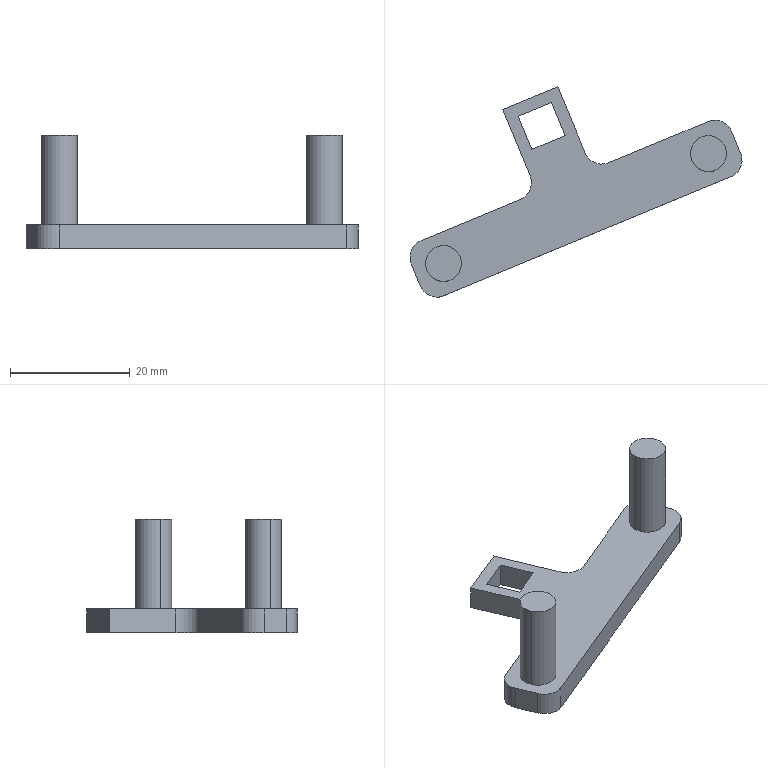Component | SolidWorks | Hanger-1 | 1 solid | 26 faces | box 55.57 x 35.2 x 19 mm | volume 3609 mm3 | plane 16 | cylinder 10 | commonest cylinder face diameters 6 x10
build123d program:
from build123d import *

# Parameters (mm, degrees)
SKETCH1_W           = 6
SKETCH1_H           = 6
BOSS_EXTRUDE1_DEPTH = 4
SKETCH2_R           = 3
BOSS_EXTRUDE2_DEPTH = 15


with BuildPart() as part:
    # Sketch1 → Boss-Extrude1 (new body)
    with BuildSketch(Plane.XY):
        with BuildLine():
            Line((-5.892, 5.811), (4.108, 5.811))
            Line((4.108, 5.811), (4.108, -4.189))
            Line((4.108, -4.189), (4.108, -6.189))
            ThreePointArc((4.108, -6.189), (4.987, -8.311), (7.108, -9.189))
            Line((7.108, -9.189), (25.108, -9.189))
            ThreePointArc((25.108, -9.189), (27.229, -10.068), (28.108, -12.189))
            Line((28.108, -12.189), (28.108, -16.189))
            ThreePointArc((28.108, -16.189), (27.229, -18.311), (25.108, -19.189))
            Line((25.108, -19.189), (-26.892, -19.189))
            ThreePointArc((-26.892, -19.189), (-29.013, -18.311), (-29.892, -16.189))
            Line((-29.892, -16.189), (-29.892, -12.189))
            ThreePointArc((-29.892, -12.189), (-29.013, -10.068), (-26.892, -9.189))
            Line((-26.892, -9.189), (-8.892, -9.189))
            ThreePointArc((-8.892, -9.189), (-6.771, -8.311), (-5.892, -6.189))
            Line((-5.892, -6.189), (-5.892, -4.189))
            Line((-5.892, -4.189), (-5.892, 5.811))
        make_face()
        with Locations((-0.8919, 0.8108)):
            Rectangle(SKETCH1_W, SKETCH1_H, mode=Mode.SUBTRACT)
    extrude(amount=BOSS_EXTRUDE1_DEPTH)

    # Sketch2 → Boss-Extrude2 (add)
    with BuildSketch(Plane(origin=(0, 0, 0), x_dir=(-1, 0, 0), z_dir=(0, 0, -1))):
        with Locations((-23.108, -14.189)):
            Circle(SKETCH2_R)
        with Locations(Location((24.892, -14.189, 0), (0, 0, 180))):
            Circle(SKETCH2_R)
    extrude(amount=BOSS_EXTRUDE2_DEPTH)


solid = part.part

# Placed as in the assembly
solid = solid.moved(Location((19.638, 31.834, 352.846), (180, 0, 157.477)))
STEP:
#1=COLOUR_RGB('',0.7922,0.8196,0.9333);
#2=FILL_AREA_STYLE_COLOUR('',#1);
#3=FILL_AREA_STYLE('',(#2));
#4=SURFACE_STYLE_FILL_AREA(#3);
#5=SURFACE_SIDE_STYLE('',(#4));
#6=SURFACE_STYLE_USAGE(.BOTH.,#5);
#7=PRESENTATION_STYLE_ASSIGNMENT((#6));
#8=CARTESIAN_POINT('',(2.001,1.158,14.482));
#9=VERTEX_POINT('',#8);
#10=CARTESIAN_POINT('',(1.783,1.067,14.482));
#11=VERTEX_POINT('',#10);
#12=CARTESIAN_POINT('',(1.892,1.113,14.482));
#13=DIRECTION('',(-0.,-0.,1.));
#14=DIRECTION('',(-0.9237,-0.383,0.));
#15=AXIS2_PLACEMENT_3D('',#12,#13,#14);
#16=CIRCLE('',#15,0.1181);
#17=EDGE_CURVE('',#9,#11,#16,.T.);
#18=ORIENTED_EDGE('',*,*,#17,.F.);
#19=CARTESIAN_POINT('',(2.001,1.158,13.892));
#20=VERTEX_POINT('',#19);
#21=CARTESIAN_POINT('',(2.001,1.158,14.482));
#22=DIRECTION('',(0.,0.,-1.));
#23=VECTOR('',#22,39.37);
#24=LINE('',#21,#23);
#25=EDGE_CURVE('',#9,#20,#24,.T.);
#26=ORIENTED_EDGE('',*,*,#25,.T.);
#27=CARTESIAN_POINT('',(1.783,1.067,13.892));
#28=VERTEX_POINT('',#27);
#29=CARTESIAN_POINT('',(1.892,1.113,13.892));
#30=DIRECTION('',(-0.,-0.,1.));
#31=DIRECTION('',(-0.9237,-0.383,0.));
#32=AXIS2_PLACEMENT_3D('',#29,#30,#31);
#33=CIRCLE('',#32,0.1181);
#34=EDGE_CURVE('',#20,#28,#33,.T.);
#35=ORIENTED_EDGE('',*,*,#34,.T.);
#36=CARTESIAN_POINT('',(1.783,1.067,14.482));
#37=DIRECTION('',(0.,0.,-1.));
#38=VECTOR('',#37,39.37);
#39=LINE('',#36,#38);
#40=EDGE_CURVE('',#11,#28,#39,.T.);
#41=ORIENTED_EDGE('',*,*,#40,.F.);
#42=EDGE_LOOP('',(#18,#26,#35,#41));
#43=FACE_OUTER_BOUND('',#42,.T.);
#44=CARTESIAN_POINT('',(1.892,1.113,14.482));
#45=DIRECTION('',(0.,0.,-1.));
#46=DIRECTION('',(-0.9237,-0.383,0.));
#47=AXIS2_PLACEMENT_3D('',#44,#45,#46);
#48=CYLINDRICAL_SURFACE('',#47,0.1181);
#49=ADVANCED_FACE('',(#43),#48,.T.);
#50=CARTESIAN_POINT('',(0.2558,0.4341,14.482));
#51=VERTEX_POINT('',#50);
#52=CARTESIAN_POINT('',(0.03764,0.3436,14.482));
#53=VERTEX_POINT('',#52);
#54=CARTESIAN_POINT('',(0.1467,0.3888,14.482));
#55=DIRECTION('',(-0.,-0.,1.));
#56=DIRECTION('',(0.9237,0.383,0.));
#57=AXIS2_PLACEMENT_3D('',#54,#55,#56);
#58=CIRCLE('',#57,0.1181);
#59=EDGE_CURVE('',#51,#53,#58,.T.);
#60=ORIENTED_EDGE('',*,*,#59,.F.);
#61=CARTESIAN_POINT('',(0.2558,0.4341,13.892));
#62=VERTEX_POINT('',#61);
#63=CARTESIAN_POINT('',(0.2558,0.4341,14.482));
#64=DIRECTION('',(0.,0.,-1.));
#65=VECTOR('',#64,39.37);
#66=LINE('',#63,#65);
#67=EDGE_CURVE('',#51,#62,#66,.T.);
#68=ORIENTED_EDGE('',*,*,#67,.T.);
#69=CARTESIAN_POINT('',(0.03764,0.3436,13.892));
#70=VERTEX_POINT('',#69);
#71=CARTESIAN_POINT('',(0.1467,0.3888,13.892));
#72=DIRECTION('',(-0.,-0.,1.));
#73=DIRECTION('',(0.9237,0.383,0.));
#74=AXIS2_PLACEMENT_3D('',#71,#72,#73);
#75=CIRCLE('',#74,0.1181);
#76=EDGE_CURVE('',#62,#70,#75,.T.);
#77=ORIENTED_EDGE('',*,*,#76,.T.);
#78=CARTESIAN_POINT('',(0.03764,0.3436,14.482));
#79=DIRECTION('',(0.,0.,-1.));
#80=VECTOR('',#79,39.37);
#81=LINE('',#78,#80);
#82=EDGE_CURVE('',#53,#70,#81,.T.);
#83=ORIENTED_EDGE('',*,*,#82,.F.);
#84=EDGE_LOOP('',(#60,#68,#77,#83));
#85=FACE_OUTER_BOUND('',#84,.T.);
#86=CARTESIAN_POINT('',(0.1467,0.3888,14.482));
#87=DIRECTION('',(0.,0.,-1.));
#88=DIRECTION('',(-0.9237,-0.383,0.));
#89=AXIS2_PLACEMENT_3D('',#86,#87,#88);
#90=CYLINDRICAL_SURFACE('',#89,0.1181);
#91=ADVANCED_FACE('',(#85),#90,.T.);
#92=CARTESIAN_POINT('',(0.8998,1.553,13.734));
#93=VERTEX_POINT('',#92);
#94=CARTESIAN_POINT('',(1.081,1.117,13.734));
#95=VERTEX_POINT('',#94);
#96=CARTESIAN_POINT('',(0.8998,1.553,13.734));
#97=DIRECTION('',(0.383,-0.9237,0.));
#98=VECTOR('',#97,39.37);
#99=LINE('',#96,#98);
#100=EDGE_CURVE('',#93,#95,#99,.T.);
#101=ORIENTED_EDGE('',*,*,#100,.T.);
#102=CARTESIAN_POINT('',(1.235,1.053,13.734));
#103=VERTEX_POINT('',#102);
#104=CARTESIAN_POINT('',(1.19,1.162,13.734));
#105=DIRECTION('',(-0.,-0.,1.));
#106=DIRECTION('',(0.9237,0.383,0.));
#107=AXIS2_PLACEMENT_3D('',#104,#105,#106);
#108=CIRCLE('',#107,0.1181);
#109=EDGE_CURVE('',#95,#103,#108,.T.);
#110=ORIENTED_EDGE('',*,*,#109,.T.);
#111=CARTESIAN_POINT('',(1.89,1.325,13.734));
#112=VERTEX_POINT('',#111);
#113=CARTESIAN_POINT('',(1.235,1.053,13.734));
#114=DIRECTION('',(0.9237,0.383,0.));
#115=VECTOR('',#114,39.37);
#116=LINE('',#113,#115);
#117=EDGE_CURVE('',#103,#112,#116,.T.);
#118=ORIENTED_EDGE('',*,*,#117,.T.);
#119=CARTESIAN_POINT('',(2.044,1.261,13.734));
#120=VERTEX_POINT('',#119);
#121=CARTESIAN_POINT('',(1.935,1.216,13.734));
#122=DIRECTION('',(0.,0.,-1.));
#123=DIRECTION('',(-0.9237,-0.383,0.));
#124=AXIS2_PLACEMENT_3D('',#121,#122,#123);
#125=CIRCLE('',#124,0.1181);
#126=EDGE_CURVE('',#112,#120,#125,.T.);
#127=ORIENTED_EDGE('',*,*,#126,.T.);
#128=CARTESIAN_POINT('',(2.104,1.115,13.734));
#129=VERTEX_POINT('',#128);
#130=CARTESIAN_POINT('',(2.044,1.261,13.734));
#131=DIRECTION('',(0.383,-0.9237,0.));
#132=VECTOR('',#131,39.37);
#133=LINE('',#130,#132);
#134=EDGE_CURVE('',#120,#129,#133,.T.);
#135=ORIENTED_EDGE('',*,*,#134,.T.);
#136=CARTESIAN_POINT('',(2.041,0.961,13.734));
#137=VERTEX_POINT('',#136);
#138=CARTESIAN_POINT('',(1.995,1.07,13.734));
#139=DIRECTION('',(0.,0.,-1.));
#140=DIRECTION('',(-0.9237,-0.383,0.));
#141=AXIS2_PLACEMENT_3D('',#138,#139,#140);
#142=CIRCLE('',#141,0.1181);
#143=EDGE_CURVE('',#129,#137,#142,.T.);
#144=ORIENTED_EDGE('',*,*,#143,.T.);
#145=CARTESIAN_POINT('',(0.1494,0.1768,13.734));
#146=VERTEX_POINT('',#145);
#147=CARTESIAN_POINT('',(2.041,0.961,13.734));
#148=DIRECTION('',(-0.9237,-0.383,-0.));
#149=VECTOR('',#148,39.37);
#150=LINE('',#147,#149);
#151=EDGE_CURVE('',#137,#146,#150,.T.);
#152=ORIENTED_EDGE('',*,*,#151,.T.);
#153=CARTESIAN_POINT('',(-0.004933,0.2407,13.734));
#154=VERTEX_POINT('',#153);
#155=CARTESIAN_POINT('',(0.1042,0.2859,13.734));
#156=DIRECTION('',(0.,0.,-1.));
#157=DIRECTION('',(0.9237,0.383,0.));
#158=AXIS2_PLACEMENT_3D('',#155,#156,#157);
#159=CIRCLE('',#158,0.1181);
#160=EDGE_CURVE('',#146,#154,#159,.T.);
#161=ORIENTED_EDGE('',*,*,#160,.T.);
#162=CARTESIAN_POINT('',(-0.06526,0.3861,13.734));
#163=VERTEX_POINT('',#162);
#164=CARTESIAN_POINT('',(-0.06526,0.3861,13.734));
#165=DIRECTION('',(-0.383,0.9237,0.));
#166=VECTOR('',#165,39.37);
#167=LINE('',#164,#166);
#168=EDGE_CURVE('',#154,#163,#167,.T.);
#169=ORIENTED_EDGE('',*,*,#168,.T.);
#170=CARTESIAN_POINT('',(-0.001396,0.5405,13.734));
#171=VERTEX_POINT('',#170);
#172=CARTESIAN_POINT('',(0.04385,0.4314,13.734));
#173=DIRECTION('',(0.,0.,-1.));
#174=DIRECTION('',(-0.9237,-0.383,0.));
#175=AXIS2_PLACEMENT_3D('',#172,#173,#174);
#176=CIRCLE('',#175,0.1181);
#177=EDGE_CURVE('',#163,#171,#176,.T.);
#178=ORIENTED_EDGE('',*,*,#177,.T.);
#179=CARTESIAN_POINT('',(0.6532,0.8119,13.734));
#180=VERTEX_POINT('',#179);
#181=CARTESIAN_POINT('',(0.6532,0.8119,13.734));
#182=DIRECTION('',(0.9237,0.383,0.));
#183=VECTOR('',#182,39.37);
#184=LINE('',#181,#183);
#185=EDGE_CURVE('',#171,#180,#184,.T.);
#186=ORIENTED_EDGE('',*,*,#185,.T.);
#187=CARTESIAN_POINT('',(0.7171,0.9663,13.734));
#188=VERTEX_POINT('',#187);
#189=CARTESIAN_POINT('',(0.608,0.921,13.734));
#190=DIRECTION('',(-0.,-0.,1.));
#191=DIRECTION('',(-0.9237,-0.383,0.));
#192=AXIS2_PLACEMENT_3D('',#189,#190,#191);
#193=CIRCLE('',#192,0.1181);
#194=EDGE_CURVE('',#180,#188,#193,.T.);
#195=ORIENTED_EDGE('',*,*,#194,.T.);
#196=CARTESIAN_POINT('',(0.5361,1.403,13.734));
#197=VERTEX_POINT('',#196);
#198=CARTESIAN_POINT('',(0.6869,1.039,13.734));
#199=DIRECTION('',(-0.383,0.9237,-0.));
#200=VECTOR('',#199,39.37);
#201=LINE('',#198,#200);
#202=EDGE_CURVE('',#188,#197,#201,.T.);
#203=ORIENTED_EDGE('',*,*,#202,.T.);
#204=CARTESIAN_POINT('',(0.8998,1.553,13.734));
#205=DIRECTION('',(0.9237,0.383,0.));
#206=VECTOR('',#205,39.37);
#207=LINE('',#204,#206);
#208=EDGE_CURVE('',#197,#93,#207,.T.);
#209=ORIENTED_EDGE('',*,*,#208,.T.);
#210=EDGE_LOOP('',(#101,#110,#118,#127,#135,#144,#152,#161,#169,#178,#186,#195,#203,#209));
#211=FACE_OUTER_BOUND('',#210,.T.);
#212=CARTESIAN_POINT('',(0.8572,1.451,13.734));
#213=VERTEX_POINT('',#212);
#214=CARTESIAN_POINT('',(0.9477,1.232,13.734));
#215=VERTEX_POINT('',#214);
#216=CARTESIAN_POINT('',(0.8572,1.451,13.734));
#217=DIRECTION('',(0.383,-0.9237,-0.));
#218=VECTOR('',#217,39.37);
#219=LINE('',#216,#218);
#220=EDGE_CURVE('',#213,#215,#219,.T.);
#221=ORIENTED_EDGE('',*,*,#220,.F.);
#222=CARTESIAN_POINT('',(0.639,1.36,13.734));
#223=VERTEX_POINT('',#222);
#224=CARTESIAN_POINT('',(0.8572,1.451,13.734));
#225=DIRECTION('',(0.9237,0.383,0.));
#226=VECTOR('',#225,39.37);
#227=LINE('',#224,#226);
#228=EDGE_CURVE('',#223,#213,#227,.T.);
#229=ORIENTED_EDGE('',*,*,#228,.F.);
#230=CARTESIAN_POINT('',(0.7295,1.142,13.734));
#231=VERTEX_POINT('',#230);
#232=CARTESIAN_POINT('',(0.639,1.36,13.734));
#233=DIRECTION('',(-0.383,0.9237,0.));
#234=VECTOR('',#233,39.37);
#235=LINE('',#232,#234);
#236=EDGE_CURVE('',#231,#223,#235,.T.);
#237=ORIENTED_EDGE('',*,*,#236,.F.);
#238=CARTESIAN_POINT('',(0.9477,1.232,13.734));
#239=DIRECTION('',(-0.9237,-0.383,-0.));
#240=VECTOR('',#239,39.37);
#241=LINE('',#238,#240);
#242=EDGE_CURVE('',#215,#231,#241,.T.);
#243=ORIENTED_EDGE('',*,*,#242,.F.);
#244=EDGE_LOOP('',(#221,#229,#237,#243));
#245=FACE_BOUND('',#244,.T.);
#246=CARTESIAN_POINT('',(1.19,1.162,13.734));
#247=DIRECTION('',(-0.,-0.,1.));
#248=DIRECTION('',(0.9237,0.383,0.));
#249=AXIS2_PLACEMENT_3D('',#246,#247,#248);
#250=PLANE('',#249);
#251=ADVANCED_FACE('',(#211,#245),#250,.F.);
#252=CARTESIAN_POINT('',(1.892,1.113,13.892));
#253=DIRECTION('',(-0.,-0.,1.));
#254=DIRECTION('',(-0.9237,-0.383,0.));
#255=AXIS2_PLACEMENT_3D('',#252,#253,#254);
#256=CIRCLE('',#255,0.1181);
#257=EDGE_CURVE('',#28,#20,#256,.T.);
#258=ORIENTED_EDGE('',*,*,#257,.F.);
#259=ORIENTED_EDGE('',*,*,#34,.F.);
#260=EDGE_LOOP('',(#258,#259));
#261=FACE_BOUND('',#260,.T.);
#262=CARTESIAN_POINT('',(0.1467,0.3888,13.892));
#263=DIRECTION('',(-0.,-0.,1.));
#264=DIRECTION('',(0.9237,0.383,0.));
#265=AXIS2_PLACEMENT_3D('',#262,#263,#264);
#266=CIRCLE('',#265,0.1181);
#267=EDGE_CURVE('',#70,#62,#266,.T.);
#268=ORIENTED_EDGE('',*,*,#267,.F.);
#269=ORIENTED_EDGE('',*,*,#76,.F.);
#270=EDGE_LOOP('',(#268,#269));
#271=FACE_BOUND('',#270,.T.);
#272=CARTESIAN_POINT('',(0.8998,1.553,13.892));
#273=VERTEX_POINT('',#272);
#274=CARTESIAN_POINT('',(1.081,1.117,13.892));
#275=VERTEX_POINT('',#274);
#276=CARTESIAN_POINT('',(1.051,1.19,13.892));
#277=DIRECTION('',(0.383,-0.9237,-0.));
#278=VECTOR('',#277,39.37);
#279=LINE('',#276,#278);
#280=EDGE_CURVE('',#273,#275,#279,.T.);
#281=ORIENTED_EDGE('',*,*,#280,.F.);
#282=CARTESIAN_POINT('',(0.5361,1.403,13.892));
#283=VERTEX_POINT('',#282);
#284=CARTESIAN_POINT('',(0.8998,1.553,13.892));
#285=DIRECTION('',(0.9237,0.383,0.));
#286=VECTOR('',#285,39.37);
#287=LINE('',#284,#286);
#288=EDGE_CURVE('',#283,#273,#287,.T.);
#289=ORIENTED_EDGE('',*,*,#288,.F.);
#290=CARTESIAN_POINT('',(0.7171,0.9663,13.892));
#291=VERTEX_POINT('',#290);
#292=CARTESIAN_POINT('',(0.5361,1.403,13.892));
#293=DIRECTION('',(-0.383,0.9237,0.));
#294=VECTOR('',#293,39.37);
#295=LINE('',#292,#294);
#296=EDGE_CURVE('',#291,#283,#295,.T.);
#297=ORIENTED_EDGE('',*,*,#296,.F.);
#298=CARTESIAN_POINT('',(0.6532,0.8119,13.892));
#299=VERTEX_POINT('',#298);
#300=CARTESIAN_POINT('',(0.608,0.921,13.892));
#301=DIRECTION('',(-0.,-0.,1.));
#302=DIRECTION('',(-0.9237,-0.383,0.));
#303=AXIS2_PLACEMENT_3D('',#300,#301,#302);
#304=CIRCLE('',#303,0.1181);
#305=EDGE_CURVE('',#299,#291,#304,.T.);
#306=ORIENTED_EDGE('',*,*,#305,.F.);
#307=CARTESIAN_POINT('',(-0.001396,0.5405,13.892));
#308=VERTEX_POINT('',#307);
#309=CARTESIAN_POINT('',(0.6532,0.8119,13.892));
#310=DIRECTION('',(0.9237,0.383,0.));
#311=VECTOR('',#310,39.37);
#312=LINE('',#309,#311);
#313=EDGE_CURVE('',#308,#299,#312,.T.);
#314=ORIENTED_EDGE('',*,*,#313,.F.);
#315=CARTESIAN_POINT('',(-0.06526,0.3861,13.892));
#316=VERTEX_POINT('',#315);
#317=CARTESIAN_POINT('',(0.04385,0.4314,13.892));
#318=DIRECTION('',(0.,0.,-1.));
#319=DIRECTION('',(-0.9237,-0.383,0.));
#320=AXIS2_PLACEMENT_3D('',#317,#318,#319);
#321=CIRCLE('',#320,0.1181);
#322=EDGE_CURVE('',#316,#308,#321,.T.);
#323=ORIENTED_EDGE('',*,*,#322,.F.);
#324=CARTESIAN_POINT('',(-0.004933,0.2407,13.892));
#325=VERTEX_POINT('',#324);
#326=CARTESIAN_POINT('',(-0.06526,0.3861,13.892));
#327=DIRECTION('',(-0.383,0.9237,0.));
#328=VECTOR('',#327,39.37);
#329=LINE('',#326,#328);
#330=EDGE_CURVE('',#325,#316,#329,.T.);
#331=ORIENTED_EDGE('',*,*,#330,.F.);
#332=CARTESIAN_POINT('',(0.1494,0.1768,13.892));
#333=VERTEX_POINT('',#332);
#334=CARTESIAN_POINT('',(0.1042,0.2859,13.892));
#335=DIRECTION('',(0.,0.,-1.));
#336=DIRECTION('',(0.9237,0.383,0.));
#337=AXIS2_PLACEMENT_3D('',#334,#335,#336);
#338=CIRCLE('',#337,0.1181);
#339=EDGE_CURVE('',#333,#325,#338,.T.);
#340=ORIENTED_EDGE('',*,*,#339,.F.);
#341=CARTESIAN_POINT('',(2.041,0.961,13.892));
#342=VERTEX_POINT('',#341);
#343=CARTESIAN_POINT('',(2.041,0.961,13.892));
#344=DIRECTION('',(-0.9237,-0.383,-0.));
#345=VECTOR('',#344,39.37);
#346=LINE('',#343,#345);
#347=EDGE_CURVE('',#342,#333,#346,.T.);
#348=ORIENTED_EDGE('',*,*,#347,.F.);
#349=CARTESIAN_POINT('',(2.104,1.115,13.892));
#350=VERTEX_POINT('',#349);
#351=CARTESIAN_POINT('',(1.995,1.07,13.892));
#352=DIRECTION('',(0.,0.,-1.));
#353=DIRECTION('',(-0.9237,-0.383,0.));
#354=AXIS2_PLACEMENT_3D('',#351,#352,#353);
#355=CIRCLE('',#354,0.1181);
#356=EDGE_CURVE('',#350,#342,#355,.T.);
#357=ORIENTED_EDGE('',*,*,#356,.F.);
#358=CARTESIAN_POINT('',(2.044,1.261,13.892));
#359=VERTEX_POINT('',#358);
#360=CARTESIAN_POINT('',(2.044,1.261,13.892));
#361=DIRECTION('',(0.383,-0.9237,0.));
#362=VECTOR('',#361,39.37);
#363=LINE('',#360,#362);
#364=EDGE_CURVE('',#359,#350,#363,.T.);
#365=ORIENTED_EDGE('',*,*,#364,.F.);
#366=CARTESIAN_POINT('',(1.89,1.325,13.892));
#367=VERTEX_POINT('',#366);
#368=CARTESIAN_POINT('',(1.935,1.216,13.892));
#369=DIRECTION('',(0.,0.,-1.));
#370=DIRECTION('',(-0.9237,-0.383,0.));
#371=AXIS2_PLACEMENT_3D('',#368,#369,#370);
#372=CIRCLE('',#371,0.1181);
#373=EDGE_CURVE('',#367,#359,#372,.T.);
#374=ORIENTED_EDGE('',*,*,#373,.F.);
#375=CARTESIAN_POINT('',(1.235,1.053,13.892));
#376=VERTEX_POINT('',#375);
#377=CARTESIAN_POINT('',(1.235,1.053,13.892));
#378=DIRECTION('',(0.9237,0.383,0.));
#379=VECTOR('',#378,39.37);
#380=LINE('',#377,#379);
#381=EDGE_CURVE('',#376,#367,#380,.T.);
#382=ORIENTED_EDGE('',*,*,#381,.F.);
#383=CARTESIAN_POINT('',(1.19,1.162,13.892));
#384=DIRECTION('',(-0.,-0.,1.));
#385=DIRECTION('',(0.9237,0.383,0.));
#386=AXIS2_PLACEMENT_3D('',#383,#384,#385);
#387=CIRCLE('',#386,0.1181);
#388=EDGE_CURVE('',#275,#376,#387,.T.);
#389=ORIENTED_EDGE('',*,*,#388,.F.);
#390=EDGE_LOOP('',(#281,#289,#297,#306,#314,#323,#331,#340,#348,#357,#365,#374,#382,#389));
#391=FACE_OUTER_BOUND('',#390,.T.);
#392=CARTESIAN_POINT('',(0.639,1.36,13.892));
#393=VERTEX_POINT('',#392);
#394=CARTESIAN_POINT('',(0.8572,1.451,13.892));
#395=VERTEX_POINT('',#394);
#396=CARTESIAN_POINT('',(0.8572,1.451,13.892));
#397=DIRECTION('',(0.9237,0.383,0.));
#398=VECTOR('',#397,39.37);
#399=LINE('',#396,#398);
#400=EDGE_CURVE('',#393,#395,#399,.T.);
#401=ORIENTED_EDGE('',*,*,#400,.T.);
#402=CARTESIAN_POINT('',(0.9477,1.232,13.892));
#403=VERTEX_POINT('',#402);
#404=CARTESIAN_POINT('',(0.8572,1.451,13.892));
#405=DIRECTION('',(0.383,-0.9237,-0.));
#406=VECTOR('',#405,39.37);
#407=LINE('',#404,#406);
#408=EDGE_CURVE('',#395,#403,#407,.T.);
#409=ORIENTED_EDGE('',*,*,#408,.T.);
#410=CARTESIAN_POINT('',(0.7295,1.142,13.892));
#411=VERTEX_POINT('',#410);
#412=CARTESIAN_POINT('',(0.9477,1.232,13.892));
#413=DIRECTION('',(-0.9237,-0.383,-0.));
#414=VECTOR('',#413,39.37);
#415=LINE('',#412,#414);
#416=EDGE_CURVE('',#403,#411,#415,.T.);
#417=ORIENTED_EDGE('',*,*,#416,.T.);
#418=CARTESIAN_POINT('',(0.639,1.36,13.892));
#419=DIRECTION('',(-0.383,0.9237,0.));
#420=VECTOR('',#419,39.37);
#421=LINE('',#418,#420);
#422=EDGE_CURVE('',#411,#393,#421,.T.);
#423=ORIENTED_EDGE('',*,*,#422,.T.);
#424=EDGE_LOOP('',(#401,#409,#417,#423));
#425=FACE_BOUND('',#424,.T.);
#426=CARTESIAN_POINT('',(1.19,1.162,13.892));
#427=DIRECTION('',(-0.,-0.,1.));
#428=DIRECTION('',(0.9237,0.383,0.));
#429=AXIS2_PLACEMENT_3D('',#426,#427,#428);
#430=PLANE('',#429);
#431=ADVANCED_FACE('',(#261,#271,#391,#425),#430,.T.);
#432=ORIENTED_EDGE('',*,*,#280,.T.);
#433=CARTESIAN_POINT('',(1.081,1.117,13.734));
#434=DIRECTION('',(-0.,-0.,1.));
#435=VECTOR('',#434,39.37);
#436=LINE('',#433,#435);
#437=EDGE_CURVE('',#95,#275,#436,.T.);
#438=ORIENTED_EDGE('',*,*,#437,.F.);
#439=ORIENTED_EDGE('',*,*,#100,.F.);
#440=CARTESIAN_POINT('',(0.8998,1.553,13.734));
#441=DIRECTION('',(-0.,-0.,1.));
#442=VECTOR('',#441,39.37);
#443=LINE('',#440,#442);
#444=EDGE_CURVE('',#93,#273,#443,.T.);
#445=ORIENTED_EDGE('',*,*,#444,.T.);
#446=EDGE_LOOP('',(#432,#438,#439,#445));
#447=FACE_OUTER_BOUND('',#446,.T.);
#448=CARTESIAN_POINT('',(1.051,1.19,13.734));
#449=DIRECTION('',(-0.9237,-0.383,-0.));
#450=DIRECTION('',(-0.383,0.9237,0.));
#451=AXIS2_PLACEMENT_3D('',#448,#449,#450);
#452=PLANE('',#451);
#453=ADVANCED_FACE('',(#447),#452,.F.);
#454=ORIENTED_EDGE('',*,*,#388,.T.);
#455=CARTESIAN_POINT('',(1.235,1.053,13.734));
#456=DIRECTION('',(-0.,-0.,1.));
#457=VECTOR('',#456,39.37);
#458=LINE('',#455,#457);
#459=EDGE_CURVE('',#103,#376,#458,.T.);
#460=ORIENTED_EDGE('',*,*,#459,.F.);
#461=ORIENTED_EDGE('',*,*,#109,.F.);
#462=ORIENTED_EDGE('',*,*,#437,.T.);
#463=EDGE_LOOP('',(#454,#460,#461,#462));
#464=FACE_OUTER_BOUND('',#463,.T.);
#465=CARTESIAN_POINT('',(1.19,1.162,13.734));
#466=DIRECTION('',(-0.,-0.,1.));
#467=DIRECTION('',(0.9237,0.383,0.));
#468=AXIS2_PLACEMENT_3D('',#465,#466,#467);
#469=CYLINDRICAL_SURFACE('',#468,0.1181);
#470=ADVANCED_FACE('',(#464),#469,.F.);
#471=ORIENTED_EDGE('',*,*,#381,.T.);
#472=CARTESIAN_POINT('',(1.89,1.325,13.734));
#473=DIRECTION('',(-0.,-0.,1.));
#474=VECTOR('',#473,39.37);
#475=LINE('',#472,#474);
#476=EDGE_CURVE('',#112,#367,#475,.T.);
#477=ORIENTED_EDGE('',*,*,#476,.F.);
#478=ORIENTED_EDGE('',*,*,#117,.F.);
#479=ORIENTED_EDGE('',*,*,#459,.T.);
#480=EDGE_LOOP('',(#471,#477,#478,#479));
#481=FACE_OUTER_BOUND('',#480,.T.);
#482=CARTESIAN_POINT('',(1.235,1.053,13.734));
#483=DIRECTION('',(0.383,-0.9237,-0.));
#484=DIRECTION('',(-0.9237,-0.383,-0.));
#485=AXIS2_PLACEMENT_3D('',#482,#483,#484);
#486=PLANE('',#485);
#487=ADVANCED_FACE('',(#481),#486,.F.);
#488=ORIENTED_EDGE('',*,*,#373,.T.);
#489=CARTESIAN_POINT('',(2.044,1.261,13.734));
#490=DIRECTION('',(-0.,-0.,1.));
#491=VECTOR('',#490,39.37);
#492=LINE('',#489,#491);
#493=EDGE_CURVE('',#120,#359,#492,.T.);
#494=ORIENTED_EDGE('',*,*,#493,.F.);
#495=ORIENTED_EDGE('',*,*,#126,.F.);
#496=ORIENTED_EDGE('',*,*,#476,.T.);
#497=EDGE_LOOP('',(#488,#494,#495,#496));
#498=FACE_OUTER_BOUND('',#497,.T.);
#499=CARTESIAN_POINT('',(1.935,1.216,13.734));
#500=DIRECTION('',(-0.,-0.,1.));
#501=DIRECTION('',(0.9237,0.383,0.));
#502=AXIS2_PLACEMENT_3D('',#499,#500,#501);
#503=CYLINDRICAL_SURFACE('',#502,0.1181);
#504=ADVANCED_FACE('',(#498),#503,.T.);
#505=ORIENTED_EDGE('',*,*,#364,.T.);
#506=CARTESIAN_POINT('',(2.104,1.115,13.734));
#507=DIRECTION('',(-0.,-0.,1.));
#508=VECTOR('',#507,39.37);
#509=LINE('',#506,#508);
#510=EDGE_CURVE('',#129,#350,#509,.T.);
#511=ORIENTED_EDGE('',*,*,#510,.F.);
#512=ORIENTED_EDGE('',*,*,#134,.F.);
#513=ORIENTED_EDGE('',*,*,#493,.T.);
#514=EDGE_LOOP('',(#505,#511,#512,#513));
#515=FACE_OUTER_BOUND('',#514,.T.);
#516=CARTESIAN_POINT('',(2.044,1.261,13.734));
#517=DIRECTION('',(-0.9237,-0.383,-0.));
#518=DIRECTION('',(-0.,-0.,1.));
#519=AXIS2_PLACEMENT_3D('',#516,#517,#518);
#520=PLANE('',#519);
#521=ADVANCED_FACE('',(#515),#520,.F.);
#522=ORIENTED_EDGE('',*,*,#356,.T.);
#523=CARTESIAN_POINT('',(2.041,0.961,13.734));
#524=DIRECTION('',(-0.,-0.,1.));
#525=VECTOR('',#524,39.37);
#526=LINE('',#523,#525);
#527=EDGE_CURVE('',#137,#342,#526,.T.);
#528=ORIENTED_EDGE('',*,*,#527,.F.);
#529=ORIENTED_EDGE('',*,*,#143,.F.);
#530=ORIENTED_EDGE('',*,*,#510,.T.);
#531=EDGE_LOOP('',(#522,#528,#529,#530));
#532=FACE_OUTER_BOUND('',#531,.T.);
#533=CARTESIAN_POINT('',(1.995,1.07,13.734));
#534=DIRECTION('',(-0.,-0.,1.));
#535=DIRECTION('',(0.9237,0.383,0.));
#536=AXIS2_PLACEMENT_3D('',#533,#534,#535);
#537=CYLINDRICAL_SURFACE('',#536,0.1181);
#538=ADVANCED_FACE('',(#532),#537,.T.);
#539=ORIENTED_EDGE('',*,*,#347,.T.);
#540=CARTESIAN_POINT('',(0.1494,0.1768,13.734));
#541=DIRECTION('',(-0.,-0.,1.));
#542=VECTOR('',#541,39.37);
#543=LINE('',#540,#542);
#544=EDGE_CURVE('',#146,#333,#543,.T.);
#545=ORIENTED_EDGE('',*,*,#544,.F.);
#546=ORIENTED_EDGE('',*,*,#151,.F.);
#547=ORIENTED_EDGE('',*,*,#527,.T.);
#548=EDGE_LOOP('',(#539,#545,#546,#547));
#549=FACE_OUTER_BOUND('',#548,.T.);
#550=CARTESIAN_POINT('',(2.041,0.961,13.734));
#551=DIRECTION('',(-0.383,0.9237,0.));
#552=DIRECTION('',(0.,0.,-1.));
#553=AXIS2_PLACEMENT_3D('',#550,#551,#552);
#554=PLANE('',#553);
#555=ADVANCED_FACE('',(#549),#554,.F.);
#556=ORIENTED_EDGE('',*,*,#339,.T.);
#557=CARTESIAN_POINT('',(-0.004933,0.2407,13.734));
#558=DIRECTION('',(-0.,-0.,1.));
#559=VECTOR('',#558,39.37);
#560=LINE('',#557,#559);
#561=EDGE_CURVE('',#154,#325,#560,.T.);
#562=ORIENTED_EDGE('',*,*,#561,.F.);
#563=ORIENTED_EDGE('',*,*,#160,.F.);
#564=ORIENTED_EDGE('',*,*,#544,.T.);
#565=EDGE_LOOP('',(#556,#562,#563,#564));
#566=FACE_OUTER_BOUND('',#565,.T.);
#567=CARTESIAN_POINT('',(0.1042,0.2859,13.734));
#568=DIRECTION('',(-0.,-0.,1.));
#569=DIRECTION('',(0.9237,0.383,0.));
#570=AXIS2_PLACEMENT_3D('',#567,#568,#569);
#571=CYLINDRICAL_SURFACE('',#570,0.1181);
#572=ADVANCED_FACE('',(#566),#571,.T.);
#573=ORIENTED_EDGE('',*,*,#330,.T.);
#574=CARTESIAN_POINT('',(-0.06526,0.3861,13.734));
#575=DIRECTION('',(-0.,-0.,1.));
#576=VECTOR('',#575,39.37);
#577=LINE('',#574,#576);
#578=EDGE_CURVE('',#163,#316,#577,.T.);
#579=ORIENTED_EDGE('',*,*,#578,.F.);
#580=ORIENTED_EDGE('',*,*,#168,.F.);
#581=ORIENTED_EDGE('',*,*,#561,.T.);
#582=EDGE_LOOP('',(#573,#579,#580,#581));
#583=FACE_OUTER_BOUND('',#582,.T.);
#584=CARTESIAN_POINT('',(-0.06526,0.3861,13.734));
#585=DIRECTION('',(0.9237,0.383,0.));
#586=DIRECTION('',(0.,0.,-1.));
#587=AXIS2_PLACEMENT_3D('',#584,#585,#586);
#588=PLANE('',#587);
#589=ADVANCED_FACE('',(#583),#588,.F.);
#590=ORIENTED_EDGE('',*,*,#322,.T.);
#591=CARTESIAN_POINT('',(-0.001396,0.5405,13.734));
#592=DIRECTION('',(-0.,-0.,1.));
#593=VECTOR('',#592,39.37);
#594=LINE('',#591,#593);
#595=EDGE_CURVE('',#171,#308,#594,.T.);
#596=ORIENTED_EDGE('',*,*,#595,.F.);
#597=ORIENTED_EDGE('',*,*,#177,.F.);
#598=ORIENTED_EDGE('',*,*,#578,.T.);
#599=EDGE_LOOP('',(#590,#596,#597,#598));
#600=FACE_OUTER_BOUND('',#599,.T.);
#601=CARTESIAN_POINT('',(0.04385,0.4314,13.734));
#602=DIRECTION('',(-0.,-0.,1.));
#603=DIRECTION('',(0.9237,0.383,0.));
#604=AXIS2_PLACEMENT_3D('',#601,#602,#603);
#605=CYLINDRICAL_SURFACE('',#604,0.1181);
#606=ADVANCED_FACE('',(#600),#605,.T.);
#607=ORIENTED_EDGE('',*,*,#313,.T.);
#608=CARTESIAN_POINT('',(0.6532,0.8119,13.734));
#609=DIRECTION('',(-0.,-0.,1.));
#610=VECTOR('',#609,39.37);
#611=LINE('',#608,#610);
#612=EDGE_CURVE('',#180,#299,#611,.T.);
#613=ORIENTED_EDGE('',*,*,#612,.F.);
#614=ORIENTED_EDGE('',*,*,#185,.F.);
#615=ORIENTED_EDGE('',*,*,#595,.T.);
#616=EDGE_LOOP('',(#607,#613,#614,#615));
#617=FACE_OUTER_BOUND('',#616,.T.);
#618=CARTESIAN_POINT('',(0.6532,0.8119,13.734));
#619=DIRECTION('',(0.383,-0.9237,0.));
#620=DIRECTION('',(-0.9237,-0.383,-0.));
#621=AXIS2_PLACEMENT_3D('',#618,#619,#620);
#622=PLANE('',#621);
#623=ADVANCED_FACE('',(#617),#622,.F.);
#624=ORIENTED_EDGE('',*,*,#305,.T.);
#625=CARTESIAN_POINT('',(0.7171,0.9663,13.734));
#626=DIRECTION('',(-0.,-0.,1.));
#627=VECTOR('',#626,39.37);
#628=LINE('',#625,#627);
#629=EDGE_CURVE('',#188,#291,#628,.T.);
#630=ORIENTED_EDGE('',*,*,#629,.F.);
#631=ORIENTED_EDGE('',*,*,#194,.F.);
#632=ORIENTED_EDGE('',*,*,#612,.T.);
#633=EDGE_LOOP('',(#624,#630,#631,#632));
#634=FACE_OUTER_BOUND('',#633,.T.);
#635=CARTESIAN_POINT('',(0.608,0.921,13.734));
#636=DIRECTION('',(-0.,-0.,1.));
#637=DIRECTION('',(0.9237,0.383,0.));
#638=AXIS2_PLACEMENT_3D('',#635,#636,#637);
#639=CYLINDRICAL_SURFACE('',#638,0.1181);
#640=ADVANCED_FACE('',(#634),#639,.F.);
#641=ORIENTED_EDGE('',*,*,#296,.T.);
#642=CARTESIAN_POINT('',(0.5361,1.403,13.734));
#643=DIRECTION('',(-0.,-0.,1.));
#644=VECTOR('',#643,39.37);
#645=LINE('',#642,#644);
#646=EDGE_CURVE('',#197,#283,#645,.T.);
#647=ORIENTED_EDGE('',*,*,#646,.F.);
#648=ORIENTED_EDGE('',*,*,#202,.F.);
#649=ORIENTED_EDGE('',*,*,#629,.T.);
#650=EDGE_LOOP('',(#641,#647,#648,#649));
#651=FACE_OUTER_BOUND('',#650,.T.);
#652=CARTESIAN_POINT('',(0.5361,1.403,13.734));
#653=DIRECTION('',(0.9237,0.383,0.));
#654=DIRECTION('',(0.,0.,-1.));
#655=AXIS2_PLACEMENT_3D('',#652,#653,#654);
#656=PLANE('',#655);
#657=ADVANCED_FACE('',(#651),#656,.F.);
#658=ORIENTED_EDGE('',*,*,#288,.T.);
#659=ORIENTED_EDGE('',*,*,#444,.F.);
#660=ORIENTED_EDGE('',*,*,#208,.F.);
#661=ORIENTED_EDGE('',*,*,#646,.T.);
#662=EDGE_LOOP('',(#658,#659,#660,#661));
#663=FACE_OUTER_BOUND('',#662,.T.);
#664=CARTESIAN_POINT('',(0.8998,1.553,13.734));
#665=DIRECTION('',(0.383,-0.9237,-0.));
#666=DIRECTION('',(-0.,-0.,1.));
#667=AXIS2_PLACEMENT_3D('',#664,#665,#666);
#668=PLANE('',#667);
#669=ADVANCED_FACE('',(#663),#668,.F.);
#670=ORIENTED_EDGE('',*,*,#408,.F.);
#671=CARTESIAN_POINT('',(0.8572,1.451,13.734));
#672=DIRECTION('',(-0.,-0.,1.));
#673=VECTOR('',#672,39.37);
#674=LINE('',#671,#673);
#675=EDGE_CURVE('',#213,#395,#674,.T.);
#676=ORIENTED_EDGE('',*,*,#675,.F.);
#677=ORIENTED_EDGE('',*,*,#220,.T.);
#678=CARTESIAN_POINT('',(0.9477,1.232,13.734));
#679=DIRECTION('',(-0.,-0.,1.));
#680=VECTOR('',#679,39.37);
#681=LINE('',#678,#680);
#682=EDGE_CURVE('',#215,#403,#681,.T.);
#683=ORIENTED_EDGE('',*,*,#682,.T.);
#684=EDGE_LOOP('',(#670,#676,#677,#683));
#685=FACE_OUTER_BOUND('',#684,.T.);
#686=CARTESIAN_POINT('',(0.8572,1.451,13.734));
#687=DIRECTION('',(-0.9237,-0.383,-0.));
#688=DIRECTION('',(-0.383,0.9237,0.));
#689=AXIS2_PLACEMENT_3D('',#686,#687,#688);
#690=PLANE('',#689);
#691=ADVANCED_FACE('',(#685),#690,.T.);
#692=ORIENTED_EDGE('',*,*,#416,.F.);
#693=ORIENTED_EDGE('',*,*,#682,.F.);
#694=ORIENTED_EDGE('',*,*,#242,.T.);
#695=CARTESIAN_POINT('',(0.7295,1.142,13.734));
#696=DIRECTION('',(-0.,-0.,1.));
#697=VECTOR('',#696,39.37);
#698=LINE('',#695,#697);
#699=EDGE_CURVE('',#231,#411,#698,.T.);
#700=ORIENTED_EDGE('',*,*,#699,.T.);
#701=EDGE_LOOP('',(#692,#693,#694,#700));
#702=FACE_OUTER_BOUND('',#701,.T.);
#703=CARTESIAN_POINT('',(0.9477,1.232,13.734));
#704=DIRECTION('',(-0.383,0.9237,0.));
#705=DIRECTION('',(0.,0.,-1.));
#706=AXIS2_PLACEMENT_3D('',#703,#704,#705);
#707=PLANE('',#706);
#708=ADVANCED_FACE('',(#702),#707,.T.);
#709=ORIENTED_EDGE('',*,*,#422,.F.);
#710=ORIENTED_EDGE('',*,*,#699,.F.);
#711=ORIENTED_EDGE('',*,*,#236,.T.);
#712=CARTESIAN_POINT('',(0.639,1.36,13.734));
#713=DIRECTION('',(-0.,-0.,1.));
#714=VECTOR('',#713,39.37);
#715=LINE('',#712,#714);
#716=EDGE_CURVE('',#223,#393,#715,.T.);
#717=ORIENTED_EDGE('',*,*,#716,.T.);
#718=EDGE_LOOP('',(#709,#710,#711,#717));
#719=FACE_OUTER_BOUND('',#718,.T.);
#720=CARTESIAN_POINT('',(0.639,1.36,13.734));
#721=DIRECTION('',(0.9237,0.383,0.));
#722=DIRECTION('',(0.383,-0.9237,-0.));
#723=AXIS2_PLACEMENT_3D('',#720,#721,#722);
#724=PLANE('',#723);
#725=ADVANCED_FACE('',(#719),#724,.T.);
#726=ORIENTED_EDGE('',*,*,#400,.F.);
#727=ORIENTED_EDGE('',*,*,#716,.F.);
#728=ORIENTED_EDGE('',*,*,#228,.T.);
#729=ORIENTED_EDGE('',*,*,#675,.T.);
#730=EDGE_LOOP('',(#726,#727,#728,#729));
#731=FACE_OUTER_BOUND('',#730,.T.);
#732=CARTESIAN_POINT('',(0.8572,1.451,13.734));
#733=DIRECTION('',(0.383,-0.9237,-0.));
#734=DIRECTION('',(-0.,-0.,1.));
#735=AXIS2_PLACEMENT_3D('',#732,#733,#734);
#736=PLANE('',#735);
#737=ADVANCED_FACE('',(#731),#736,.T.);
#738=ORIENTED_EDGE('',*,*,#67,.F.);
#739=CARTESIAN_POINT('',(0.1467,0.3888,14.482));
#740=DIRECTION('',(-0.,-0.,1.));
#741=DIRECTION('',(0.9237,0.383,0.));
#742=AXIS2_PLACEMENT_3D('',#739,#740,#741);
#743=CIRCLE('',#742,0.1181);
#744=EDGE_CURVE('',#53,#51,#743,.T.);
#745=ORIENTED_EDGE('',*,*,#744,.F.);
#746=ORIENTED_EDGE('',*,*,#82,.T.);
#747=ORIENTED_EDGE('',*,*,#267,.T.);
#748=EDGE_LOOP('',(#738,#745,#746,#747));
#749=FACE_OUTER_BOUND('',#748,.T.);
#750=CARTESIAN_POINT('',(0.1467,0.3888,14.482));
#751=DIRECTION('',(0.,0.,-1.));
#752=DIRECTION('',(-0.9237,-0.383,0.));
#753=AXIS2_PLACEMENT_3D('',#750,#751,#752);
#754=CYLINDRICAL_SURFACE('',#753,0.1181);
#755=ADVANCED_FACE('',(#749),#754,.T.);
#756=ORIENTED_EDGE('',*,*,#744,.T.);
#757=ORIENTED_EDGE('',*,*,#59,.T.);
#758=EDGE_LOOP('',(#756,#757));
#759=FACE_OUTER_BOUND('',#758,.T.);
#760=CARTESIAN_POINT('',(0.1467,0.3888,14.482));
#761=DIRECTION('',(-0.,-0.,1.));
#762=DIRECTION('',(0.9237,0.383,0.));
#763=AXIS2_PLACEMENT_3D('',#760,#761,#762);
#764=PLANE('',#763);
#765=ADVANCED_FACE('',(#759),#764,.T.);
#766=ORIENTED_EDGE('',*,*,#25,.F.);
#767=CARTESIAN_POINT('',(1.892,1.113,14.482));
#768=DIRECTION('',(-0.,-0.,1.));
#769=DIRECTION('',(-0.9237,-0.383,0.));
#770=AXIS2_PLACEMENT_3D('',#767,#768,#769);
#771=CIRCLE('',#770,0.1181);
#772=EDGE_CURVE('',#11,#9,#771,.T.);
#773=ORIENTED_EDGE('',*,*,#772,.F.);
#774=ORIENTED_EDGE('',*,*,#40,.T.);
#775=ORIENTED_EDGE('',*,*,#257,.T.);
#776=EDGE_LOOP('',(#766,#773,#774,#775));
#777=FACE_OUTER_BOUND('',#776,.T.);
#778=CARTESIAN_POINT('',(1.892,1.113,14.482));
#779=DIRECTION('',(0.,0.,-1.));
#780=DIRECTION('',(-0.9237,-0.383,0.));
#781=AXIS2_PLACEMENT_3D('',#778,#779,#780);
#782=CYLINDRICAL_SURFACE('',#781,0.1181);
#783=ADVANCED_FACE('',(#777),#782,.T.);
#784=ORIENTED_EDGE('',*,*,#772,.T.);
#785=ORIENTED_EDGE('',*,*,#17,.T.);
#786=EDGE_LOOP('',(#784,#785));
#787=FACE_OUTER_BOUND('',#786,.T.);
#788=CARTESIAN_POINT('',(1.892,1.113,14.482));
#789=DIRECTION('',(0.,0.,-1.));
#790=DIRECTION('',(-0.9237,-0.383,-0.));
#791=AXIS2_PLACEMENT_3D('',#788,#789,#790);
#792=PLANE('',#791);
#793=ADVANCED_FACE('',(#787),#792,.F.);
#794=CLOSED_SHELL('',(#49,#91,#251,#431,#453,#470,#487,#504,#521,#538,#555,#572,#589,#606,#623,#640,#657,#669,#691,#708,#725,#737,#755,#765,#783,#793));
#795=MANIFOLD_SOLID_BREP('',#794);
#796=STYLED_ITEM('',(#7),#795);
#797=PRESENTATION_LAYER_ASSIGNMENT('','',(#796));
#798=(LENGTH_UNIT()NAMED_UNIT(*)SI_UNIT($,.METRE.));
#799=LENGTH_MEASURE_WITH_UNIT(LENGTH_MEASURE(0.0254),#798);
#800=DIMENSIONAL_EXPONENTS(1.,0.,0.,0.,0.,0.,0.);
#801=(CONVERSION_BASED_UNIT('',#799)LENGTH_UNIT()NAMED_UNIT(#800));
#802=UNCERTAINTY_MEASURE_WITH_UNIT(LENGTH_MEASURE(0.00001),#801,'','');
#803=(NAMED_UNIT(*)PLANE_ANGLE_UNIT()SI_UNIT($,.RADIAN.));
#804=(NAMED_UNIT(*)SI_UNIT($,.STERADIAN.)SOLID_ANGLE_UNIT());
#805=(GEOMETRIC_REPRESENTATION_CONTEXT(3)GLOBAL_UNCERTAINTY_ASSIGNED_CONTEXT((#802))GLOBAL_UNIT_ASSIGNED_CONTEXT((#801,#803,#804))REPRESENTATION_CONTEXT('',''));
#806=MECHANICAL_DESIGN_GEOMETRIC_PRESENTATION_REPRESENTATION('',(#796),#805);
#807=CARTESIAN_POINT('',(0.,0.,0.));
#808=DIRECTION('',(0.,0.,1.));
#809=DIRECTION('',(1.,0.,0.));
#810=AXIS2_PLACEMENT_3D('',#807,#808,#809);
#811=(LENGTH_UNIT()NAMED_UNIT(*)SI_UNIT($,.METRE.));
#812=LENGTH_MEASURE_WITH_UNIT(LENGTH_MEASURE(0.0254),#811);
#813=DIMENSIONAL_EXPONENTS(1.,0.,0.,0.,0.,0.,0.);
#814=(CONVERSION_BASED_UNIT('',#812)LENGTH_UNIT()NAMED_UNIT(#813));
#815=UNCERTAINTY_MEASURE_WITH_UNIT(LENGTH_MEASURE(0.00001),#814,'','');
#816=(NAMED_UNIT(*)PLANE_ANGLE_UNIT()SI_UNIT($,.RADIAN.));
#817=(NAMED_UNIT(*)SI_UNIT($,.STERADIAN.)SOLID_ANGLE_UNIT());
#818=(GEOMETRIC_REPRESENTATION_CONTEXT(3)GLOBAL_UNCERTAINTY_ASSIGNED_CONTEXT((#815))GLOBAL_UNIT_ASSIGNED_CONTEXT((#814,#816,#817))REPRESENTATION_CONTEXT('',''));
#819=ADVANCED_BREP_SHAPE_REPRESENTATION('',(#795,#810),#818);